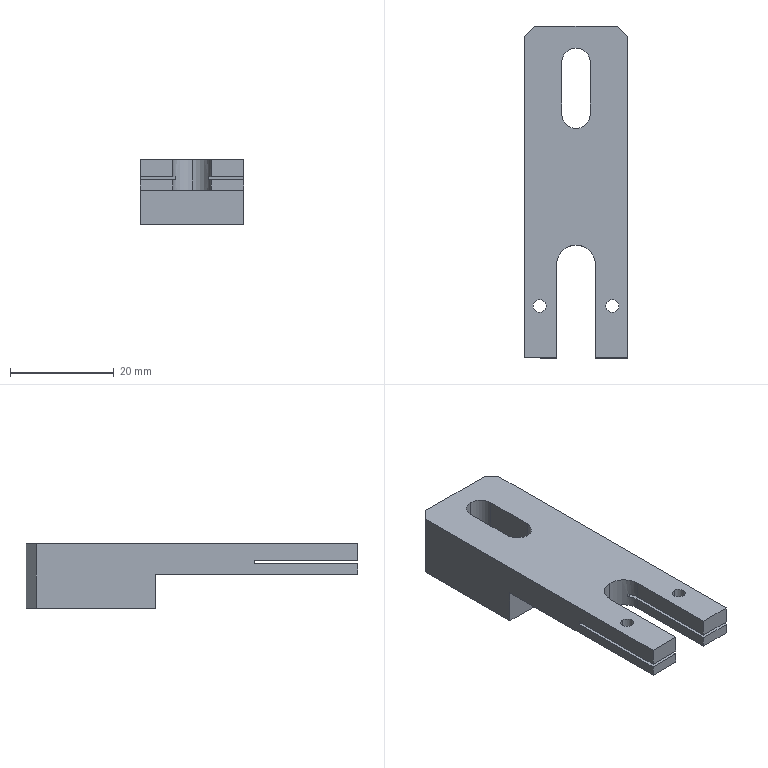Component | SolidWorks | 2018SOLIDWORKS1400000006-1 | 1 solid | 38 faces | box 20 x 64 x 12.5 mm | volume 8688 mm3 | plane 25 | cylinder 13 | commonest cylinder face diameters 2.5 x8 5.5 x3 7.5 x2 | material 45 Steel
build123d program:
from build123d import *

# Parameters (mm, degrees)
SKETCH1_W           = 64
SKETCH1_H           = 20
BOSS_EXTRUDE1_DEPTH = 12.5
SKETCH3_W           = 39
SKETCH3_H           = 20
CUT_EXTRUDE2_DEPTH  = 6.6
CHAMFER3_SIZE       = 2
CUT_EXTRUDE5_DEPTH  = 20
CUT_EXTRUDE6_DEPTH  = 36.781
M3_TAPPED_HOLE1_D   = 2.5
SKETCH12_W          = 20
SKETCH12_H          = 0.6
CUT_EXTRUDE8_DEPTH  = 40.752


with BuildPart() as part:
    # Sketch1 → Boss-Extrude1 (new body)
    with BuildSketch(Plane.XY):
        Rectangle(SKETCH1_W, SKETCH1_H)
    extrude(amount=BOSS_EXTRUDE1_DEPTH)

    # Sketch3 → Cut-Extrude2 (cut)
    with BuildSketch(Plane(origin=(0, 0, 0), x_dir=(-1, 0, 0), z_dir=(0, 0, -1))):
        with Locations((12.5, 0)):
            Rectangle(SKETCH3_W, SKETCH3_H)
    extrude(amount=-CUT_EXTRUDE2_DEPTH, mode=Mode.SUBTRACT)

    # Chamfer3
    chamfer3_edges = [part.edges().sort_by_distance(p)[0] for p in [
        (32, -10, 6.25),
        (32, 10, 6.25),
    ]]
    chamfer(chamfer3_edges, length=CHAMFER3_SIZE)

    # Sketch7 → Cut-Extrude5 (cut)
    with BuildSketch(Plane.XY.offset(12.5)):
        with BuildLine():
            Line((-32, 3.75), (-14, 3.75))
            ThreePointArc((-14, 3.75), (-10.25, 0), (-14, -3.75))
            Line((-14, -3.75), (-32, -3.75))
            ThreePointArc((-32, -3.75), (-35.75, 0), (-32, 3.75))
        make_face()
    extrude(amount=-CUT_EXTRUDE5_DEPTH, mode=Mode.SUBTRACT)

    # Sketch8 → Cut-Extrude6 (cut, through all)
    with BuildSketch(Plane.XY.offset(12.5)):
        with BuildLine():
            Line((15, 2.75), (25, 2.75))
            ThreePointArc((25, 2.75), (27.75, 0), (25, -2.75))
            Line((25, -2.75), (15, -2.75))
            ThreePointArc((15, -2.75), (12.25, 0), (15, 2.75))
        make_face()
    extrude(amount=-CUT_EXTRUDE6_DEPTH, mode=Mode.SUBTRACT)

    # M3 Tapped Hole1 (through all)
    with Locations(Plane.XY.offset(12.5)):
        with Locations((-22, 7), (-22, -7)):
            Hole(M3_TAPPED_HOLE1_D / 2)

    # Sketch12 → Cut-Extrude8 (cut, through all)
    with BuildSketch(Plane.XZ.offset(10)):
        with Locations((-22, 8.9)):
            Rectangle(SKETCH12_W, SKETCH12_H)
    extrude(amount=-CUT_EXTRUDE8_DEPTH, mode=Mode.SUBTRACT)


solid = part.part

# Placed as in the assembly
solid = solid.moved(Location((99.712, -74.5, 211), (0, 0, 90)))